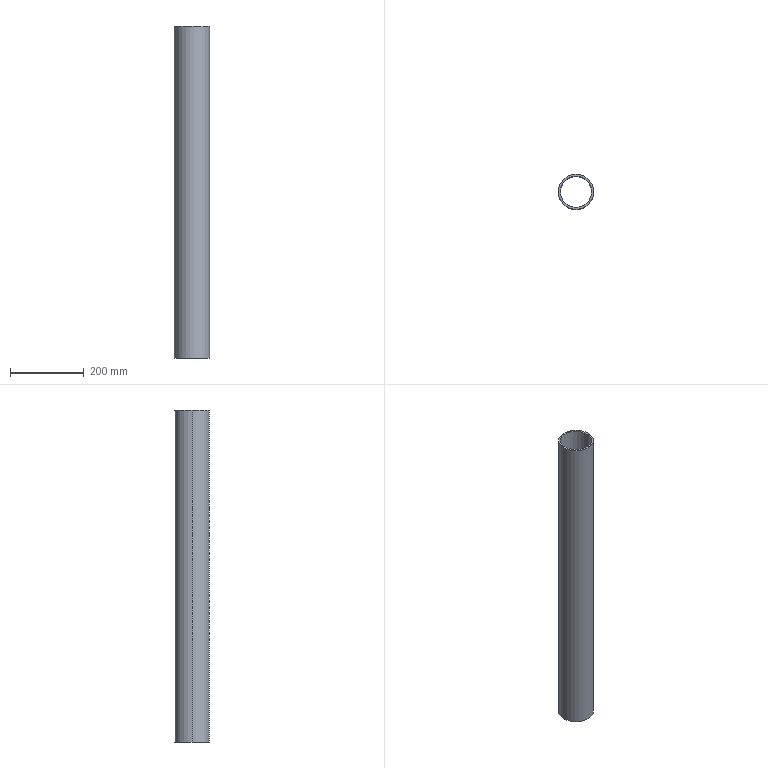Component | SolidWorks | CylinderWall1-1 | 1 solid | 6 faces | box 95 x 95 x 900 mm | volume 1272345 mm3 | cylinder 4 | plane 2 | commonest cylinder face diameters 85 x2 95 x2 | material 201 Annealed Stainless Steel (SS)
build123d program:
from build123d import *

# Parameters (mm, degrees)
SKETCH1_R           = 47.5
SKETCH1_R_2         = 42.5
BOSS_EXTRUDE1_DEPTH = 900


with BuildPart() as part:
    # Sketch1 → Boss-Extrude1 (new body)
    with BuildSketch(Plane.XY):
        Circle(SKETCH1_R)
        Circle(SKETCH1_R_2, mode=Mode.SUBTRACT)
    extrude(amount=BOSS_EXTRUDE1_DEPTH)


solid = part.part

# Placed as in the assembly
solid = solid.moved(Location((-7.456, 2.584, -375), (0, 0, 0)))
STEP:
#1=COLOUR_RGB('',0.7922,0.8196,0.9333);
#2=FILL_AREA_STYLE_COLOUR('',#1);
#3=FILL_AREA_STYLE('',(#2));
#4=SURFACE_STYLE_FILL_AREA(#3);
#5=SURFACE_SIDE_STYLE('',(#4));
#6=SURFACE_STYLE_USAGE(.BOTH.,#5);
#7=PRESENTATION_STYLE_ASSIGNMENT((#6));
#8=CARTESIAN_POINT('',(-1.967,0.1017,20.669));
#9=VERTEX_POINT('',#8);
#10=CARTESIAN_POINT('',(1.38,0.1017,20.669));
#11=VERTEX_POINT('',#10);
#12=CARTESIAN_POINT('',(-0.2935,0.1017,20.669));
#13=DIRECTION('',(0.,0.,1.));
#14=DIRECTION('',(1.,0.,0.));
#15=AXIS2_PLACEMENT_3D('',#12,#13,#14);
#16=CIRCLE('',#15,1.673);
#17=EDGE_CURVE('',#9,#11,#16,.T.);
#18=ORIENTED_EDGE('',*,*,#17,.T.);
#19=CARTESIAN_POINT('',(1.38,0.1017,-14.764));
#20=VERTEX_POINT('',#19);
#21=CARTESIAN_POINT('',(1.38,0.1017,20.669));
#22=DIRECTION('',(0.,0.,-1.));
#23=VECTOR('',#22,39.37);
#24=LINE('',#21,#23);
#25=EDGE_CURVE('',#11,#20,#24,.T.);
#26=ORIENTED_EDGE('',*,*,#25,.T.);
#27=CARTESIAN_POINT('',(-1.967,0.1017,-14.764));
#28=VERTEX_POINT('',#27);
#29=CARTESIAN_POINT('',(-0.2935,0.1017,-14.764));
#30=DIRECTION('',(0.,0.,1.));
#31=DIRECTION('',(1.,0.,0.));
#32=AXIS2_PLACEMENT_3D('',#29,#30,#31);
#33=CIRCLE('',#32,1.673);
#34=EDGE_CURVE('',#28,#20,#33,.T.);
#35=ORIENTED_EDGE('',*,*,#34,.F.);
#36=CARTESIAN_POINT('',(-1.967,0.1017,20.669));
#37=DIRECTION('',(0.,0.,-1.));
#38=VECTOR('',#37,39.37);
#39=LINE('',#36,#38);
#40=EDGE_CURVE('',#9,#28,#39,.T.);
#41=ORIENTED_EDGE('',*,*,#40,.F.);
#42=EDGE_LOOP('',(#18,#26,#35,#41));
#43=FACE_OUTER_BOUND('',#42,.T.);
#44=CARTESIAN_POINT('',(-0.2935,0.1017,20.669));
#45=DIRECTION('',(0.,0.,-1.));
#46=DIRECTION('',(-1.,0.,0.));
#47=AXIS2_PLACEMENT_3D('',#44,#45,#46);
#48=CYLINDRICAL_SURFACE('',#47,1.673);
#49=ADVANCED_FACE('',(#43),#48,.F.);
#50=CARTESIAN_POINT('',(1.577,0.1017,20.669));
#51=VERTEX_POINT('',#50);
#52=CARTESIAN_POINT('',(-2.164,0.1017,20.669));
#53=VERTEX_POINT('',#52);
#54=CARTESIAN_POINT('',(-0.2935,0.1017,20.669));
#55=DIRECTION('',(0.,0.,1.));
#56=DIRECTION('',(1.,0.,0.));
#57=AXIS2_PLACEMENT_3D('',#54,#55,#56);
#58=CIRCLE('',#57,1.87);
#59=EDGE_CURVE('',#51,#53,#58,.T.);
#60=ORIENTED_EDGE('',*,*,#59,.F.);
#61=CARTESIAN_POINT('',(1.577,0.1017,-14.764));
#62=VERTEX_POINT('',#61);
#63=CARTESIAN_POINT('',(1.577,0.1017,20.669));
#64=DIRECTION('',(0.,0.,-1.));
#65=VECTOR('',#64,39.37);
#66=LINE('',#63,#65);
#67=EDGE_CURVE('',#51,#62,#66,.T.);
#68=ORIENTED_EDGE('',*,*,#67,.T.);
#69=CARTESIAN_POINT('',(-2.164,0.1017,-14.764));
#70=VERTEX_POINT('',#69);
#71=CARTESIAN_POINT('',(-0.2935,0.1017,-14.764));
#72=DIRECTION('',(0.,0.,1.));
#73=DIRECTION('',(1.,0.,0.));
#74=AXIS2_PLACEMENT_3D('',#71,#72,#73);
#75=CIRCLE('',#74,1.87);
#76=EDGE_CURVE('',#62,#70,#75,.T.);
#77=ORIENTED_EDGE('',*,*,#76,.T.);
#78=CARTESIAN_POINT('',(-2.164,0.1017,20.669));
#79=DIRECTION('',(0.,0.,-1.));
#80=VECTOR('',#79,39.37);
#81=LINE('',#78,#80);
#82=EDGE_CURVE('',#53,#70,#81,.T.);
#83=ORIENTED_EDGE('',*,*,#82,.F.);
#84=EDGE_LOOP('',(#60,#68,#77,#83));
#85=FACE_OUTER_BOUND('',#84,.T.);
#86=CARTESIAN_POINT('',(-0.2935,0.1017,20.669));
#87=DIRECTION('',(0.,0.,-1.));
#88=DIRECTION('',(-1.,0.,0.));
#89=AXIS2_PLACEMENT_3D('',#86,#87,#88);
#90=CYLINDRICAL_SURFACE('',#89,1.87);
#91=ADVANCED_FACE('',(#85),#90,.T.);
#92=CARTESIAN_POINT('',(-0.2935,0.1017,20.669));
#93=DIRECTION('',(0.,0.,1.));
#94=DIRECTION('',(1.,0.,0.));
#95=AXIS2_PLACEMENT_3D('',#92,#93,#94);
#96=CIRCLE('',#95,1.87);
#97=EDGE_CURVE('',#53,#51,#96,.T.);
#98=ORIENTED_EDGE('',*,*,#97,.T.);
#99=ORIENTED_EDGE('',*,*,#59,.T.);
#100=EDGE_LOOP('',(#98,#99));
#101=FACE_OUTER_BOUND('',#100,.T.);
#102=ORIENTED_EDGE('',*,*,#17,.F.);
#103=CARTESIAN_POINT('',(-0.2935,0.1017,20.669));
#104=DIRECTION('',(0.,0.,1.));
#105=DIRECTION('',(1.,0.,0.));
#106=AXIS2_PLACEMENT_3D('',#103,#104,#105);
#107=CIRCLE('',#106,1.673);
#108=EDGE_CURVE('',#11,#9,#107,.T.);
#109=ORIENTED_EDGE('',*,*,#108,.F.);
#110=EDGE_LOOP('',(#102,#109));
#111=FACE_BOUND('',#110,.T.);
#112=CARTESIAN_POINT('',(-0.2935,0.1017,20.669));
#113=DIRECTION('',(0.,0.,1.));
#114=DIRECTION('',(1.,0.,0.));
#115=AXIS2_PLACEMENT_3D('',#112,#113,#114);
#116=PLANE('',#115);
#117=ADVANCED_FACE('',(#101,#111),#116,.T.);
#118=CARTESIAN_POINT('',(-0.2935,0.1017,-14.764));
#119=DIRECTION('',(0.,0.,1.));
#120=DIRECTION('',(1.,0.,0.));
#121=AXIS2_PLACEMENT_3D('',#118,#119,#120);
#122=CIRCLE('',#121,1.87);
#123=EDGE_CURVE('',#70,#62,#122,.T.);
#124=ORIENTED_EDGE('',*,*,#123,.F.);
#125=ORIENTED_EDGE('',*,*,#76,.F.);
#126=EDGE_LOOP('',(#124,#125));
#127=FACE_OUTER_BOUND('',#126,.T.);
#128=ORIENTED_EDGE('',*,*,#34,.T.);
#129=CARTESIAN_POINT('',(-0.2935,0.1017,-14.764));
#130=DIRECTION('',(0.,0.,1.));
#131=DIRECTION('',(1.,0.,0.));
#132=AXIS2_PLACEMENT_3D('',#129,#130,#131);
#133=CIRCLE('',#132,1.673);
#134=EDGE_CURVE('',#20,#28,#133,.T.);
#135=ORIENTED_EDGE('',*,*,#134,.T.);
#136=EDGE_LOOP('',(#128,#135));
#137=FACE_BOUND('',#136,.T.);
#138=CARTESIAN_POINT('',(-0.2935,0.1017,-14.764));
#139=DIRECTION('',(0.,0.,1.));
#140=DIRECTION('',(1.,0.,0.));
#141=AXIS2_PLACEMENT_3D('',#138,#139,#140);
#142=PLANE('',#141);
#143=ADVANCED_FACE('',(#127,#137),#142,.F.);
#144=ORIENTED_EDGE('',*,*,#67,.F.);
#145=ORIENTED_EDGE('',*,*,#97,.F.);
#146=ORIENTED_EDGE('',*,*,#82,.T.);
#147=ORIENTED_EDGE('',*,*,#123,.T.);
#148=EDGE_LOOP('',(#144,#145,#146,#147));
#149=FACE_OUTER_BOUND('',#148,.T.);
#150=CARTESIAN_POINT('',(-0.2935,0.1017,20.669));
#151=DIRECTION('',(0.,0.,-1.));
#152=DIRECTION('',(-1.,0.,0.));
#153=AXIS2_PLACEMENT_3D('',#150,#151,#152);
#154=CYLINDRICAL_SURFACE('',#153,1.87);
#155=ADVANCED_FACE('',(#149),#154,.T.);
#156=ORIENTED_EDGE('',*,*,#25,.F.);
#157=ORIENTED_EDGE('',*,*,#108,.T.);
#158=ORIENTED_EDGE('',*,*,#40,.T.);
#159=ORIENTED_EDGE('',*,*,#134,.F.);
#160=EDGE_LOOP('',(#156,#157,#158,#159));
#161=FACE_OUTER_BOUND('',#160,.T.);
#162=CARTESIAN_POINT('',(-0.2935,0.1017,20.669));
#163=DIRECTION('',(0.,0.,-1.));
#164=DIRECTION('',(-1.,0.,0.));
#165=AXIS2_PLACEMENT_3D('',#162,#163,#164);
#166=CYLINDRICAL_SURFACE('',#165,1.673);
#167=ADVANCED_FACE('',(#161),#166,.F.);
#168=CLOSED_SHELL('',(#49,#91,#117,#143,#155,#167));
#169=MANIFOLD_SOLID_BREP('',#168);
#170=STYLED_ITEM('',(#7),#169);
#171=PRESENTATION_LAYER_ASSIGNMENT('','',(#170));
#172=(LENGTH_UNIT()NAMED_UNIT(*)SI_UNIT($,.METRE.));
#173=LENGTH_MEASURE_WITH_UNIT(LENGTH_MEASURE(0.0254),#172);
#174=DIMENSIONAL_EXPONENTS(1.,0.,0.,0.,0.,0.,0.);
#175=(CONVERSION_BASED_UNIT('',#173)LENGTH_UNIT()NAMED_UNIT(#174));
#176=UNCERTAINTY_MEASURE_WITH_UNIT(LENGTH_MEASURE(0.00001),#175,'','');
#177=(NAMED_UNIT(*)PLANE_ANGLE_UNIT()SI_UNIT($,.RADIAN.));
#178=(NAMED_UNIT(*)SI_UNIT($,.STERADIAN.)SOLID_ANGLE_UNIT());
#179=(GEOMETRIC_REPRESENTATION_CONTEXT(3)GLOBAL_UNCERTAINTY_ASSIGNED_CONTEXT((#176))GLOBAL_UNIT_ASSIGNED_CONTEXT((#175,#177,#178))REPRESENTATION_CONTEXT('',''));
#180=MECHANICAL_DESIGN_GEOMETRIC_PRESENTATION_REPRESENTATION('',(#170),#179);
#181=CARTESIAN_POINT('',(0.,0.,0.));
#182=DIRECTION('',(0.,0.,1.));
#183=DIRECTION('',(1.,0.,0.));
#184=AXIS2_PLACEMENT_3D('',#181,#182,#183);
#185=(LENGTH_UNIT()NAMED_UNIT(*)SI_UNIT($,.METRE.));
#186=LENGTH_MEASURE_WITH_UNIT(LENGTH_MEASURE(0.0254),#185);
#187=DIMENSIONAL_EXPONENTS(1.,0.,0.,0.,0.,0.,0.);
#188=(CONVERSION_BASED_UNIT('',#186)LENGTH_UNIT()NAMED_UNIT(#187));
#189=UNCERTAINTY_MEASURE_WITH_UNIT(LENGTH_MEASURE(0.00001),#188,'','');
#190=(NAMED_UNIT(*)PLANE_ANGLE_UNIT()SI_UNIT($,.RADIAN.));
#191=(NAMED_UNIT(*)SI_UNIT($,.STERADIAN.)SOLID_ANGLE_UNIT());
#192=(GEOMETRIC_REPRESENTATION_CONTEXT(3)GLOBAL_UNCERTAINTY_ASSIGNED_CONTEXT((#189))GLOBAL_UNIT_ASSIGNED_CONTEXT((#188,#190,#191))REPRESENTATION_CONTEXT('',''));
#193=ADVANCED_BREP_SHAPE_REPRESENTATION('',(#169,#184),#192);